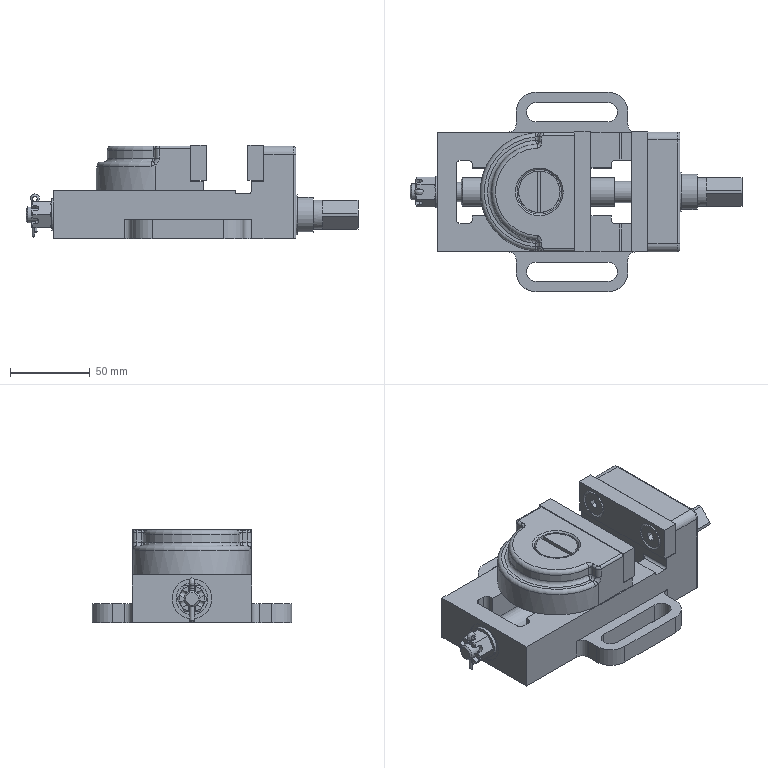Assembly | NX | mm | 14 component files | 14 solids | 311 faces | box 208 x 125 x 58.5 mm | volume 479498 mm3 | plane 160 | cylinder 90 | cone 39 | torus 13 | spline 9 | commonest cylinder face diameters 3 x13 10 x10 8 x8 6 x8 12 x6 25 x6 3.8 x6 18 x5
Bill of materials:
unnamed part 1 | 1 |  | Rectangular frame-like block. It has a large rectangular through-window, a thin base plate with two opposing mounting tabs that carry slots, and a raised end block with holes.
unnamed part 2 | 1 |  | Short headed pin or screw-like part. It has a large cylindrical head with a straight slot across it and a smaller cylindrical shank with a chamfered end.
unnamed part 3 | 2 |  | Plain rectangular bar or block with two round through-holes through its broad face, one near each end.
unnamed part 4 | 1 |  | Block with a T-shaped base: a rectangular block on a wider flanged foot, with a large horizontal through-bore and a cylindrical boss on top that has a smaller vertical bore.
unnamed part 5 | 1 |  | Hexagonal nut-like body with a central through-bore and several radial slots with rounded ends cut into one end face, in the style of a castellated or slotted nut.
unnamed part 6 | 1 |  | Thin flat annular ring (washer-like): a circular disc with a concentric through-hole.
unnamed part 7 | 1 |  | Bracket or housing block with one rounded (semicircular) end and one rectangular end. It has a stepped central bore, a stepped arc-shaped ledge around the rounded end, a flat flange along one side, and two holes on a side face.
unnamed part 8 | 4 |  | Countersunk-head pin or fastener-like part: a conical (flat-countersunk) head on a plain cylindrical shank with a chamfered tip.
unnamed part 9 | 1 |  | Split-pin-like part: a looped eye head with two parallel legs of unequal length that end in angled tips.
unnamed part 10 | 1 |  | Long stepped cylindrical shaft. It has several diameter steps, a reduced neck or groove, a raised collar, a square-section end, and a small cross hole near the opposite, narrow end.
Mates:
1. fix | 1 1 component
2. touch align | 6 1 face | 1 1 face
3. touch align | 6 1 face | 1 1 face
4. angle | 6 1 face | assembly datumplane
5. touch align | 3 1 face | assembly datumplane
6. touch align | 3 1 face | 1 1 face
7. distance | 3 1 face | 1 1 face
8. touch align | 2 1 face | 1 1 face
9. touch align | 2 1 face | 1 1 face
10. touch align | 2 1 face | 1 1 face
11. touch align | 2 2 face | 3 1 face
12. touch align | 2 2 face | 3 1 face
13. touch align | 2 2 face | 3 1 face
14. touch align | 10 4 face | 2 2 face
15. touch align | 10 4 face | 2 2 face
16. touch align | 10 3 face | 2 2 face
17. touch align | 10 3 face | 2 2 face
18. touch align | 10 1 face | 2 1 face
19. touch align | 10 1 face | 2 1 face
20. touch align | 10 2 face | 1 1 face
21. touch align | 10 2 face | 2 1 face
22. touch align | 7 1 face | 6 1 face
23. touch align | 7 1 face | 1 1 face
24. touch align | 8 1 face | 6 1 face
25. touch align | 8 1 face | 7 1 face
26. touch align | 9 1 face | 6 1 face
27. touch align | 5 1 face | 3 1 face
28. touch align | 5 1 face | 6 1 face
29. touch align | 4 1 face | 3 1 face
30. touch align | 4 1 face | 5 1 face
31. parallel | 4 1 face | assembly datumplane